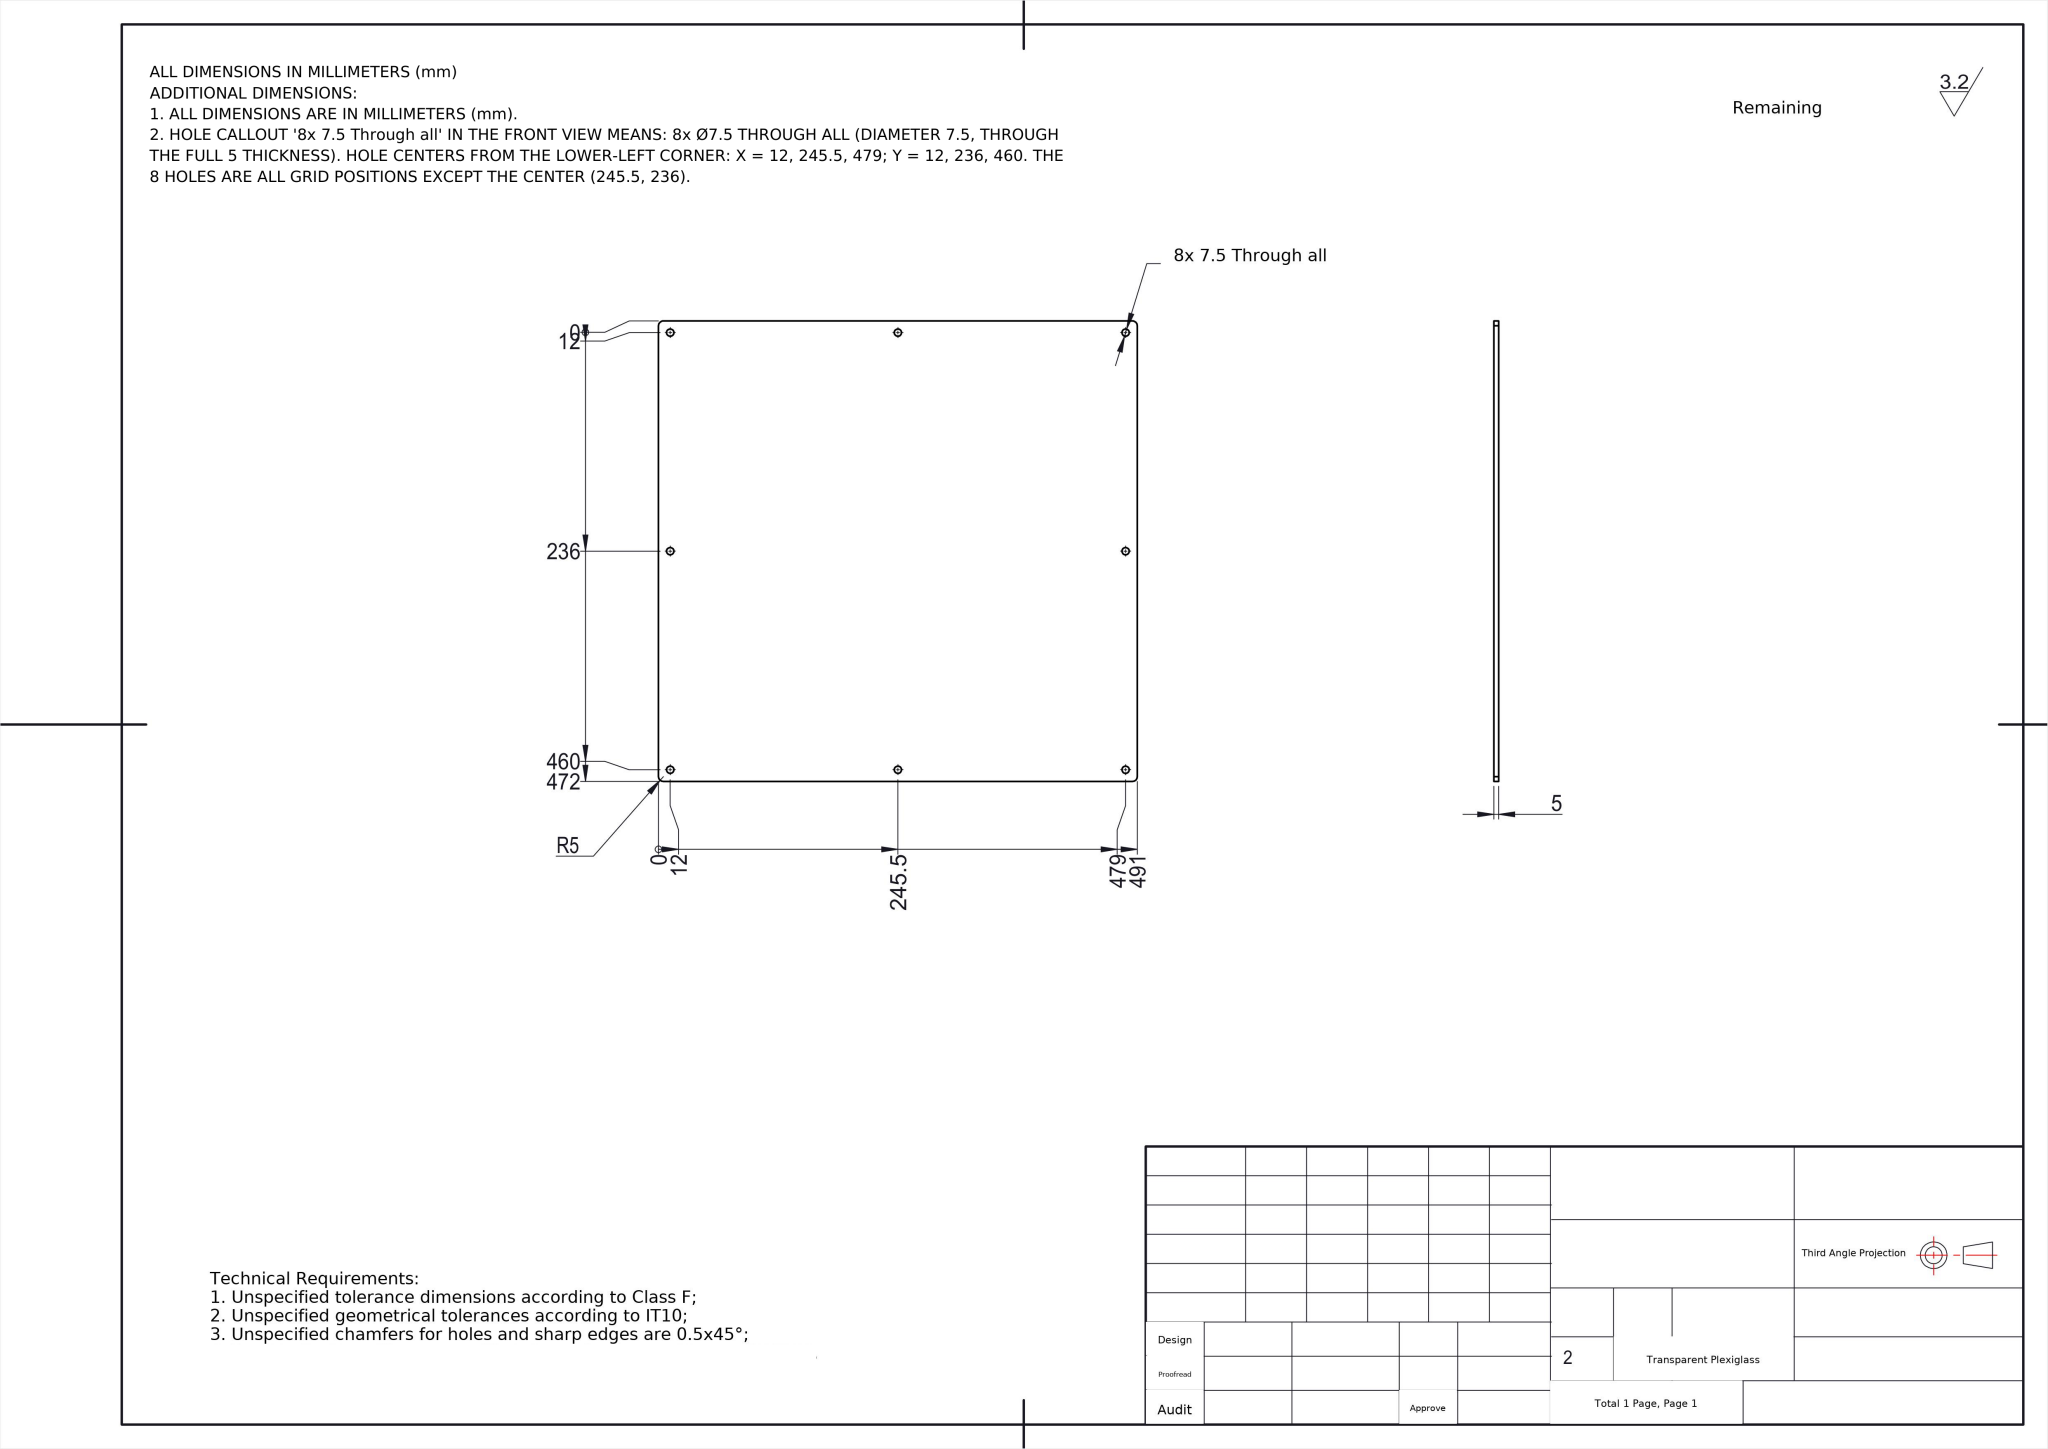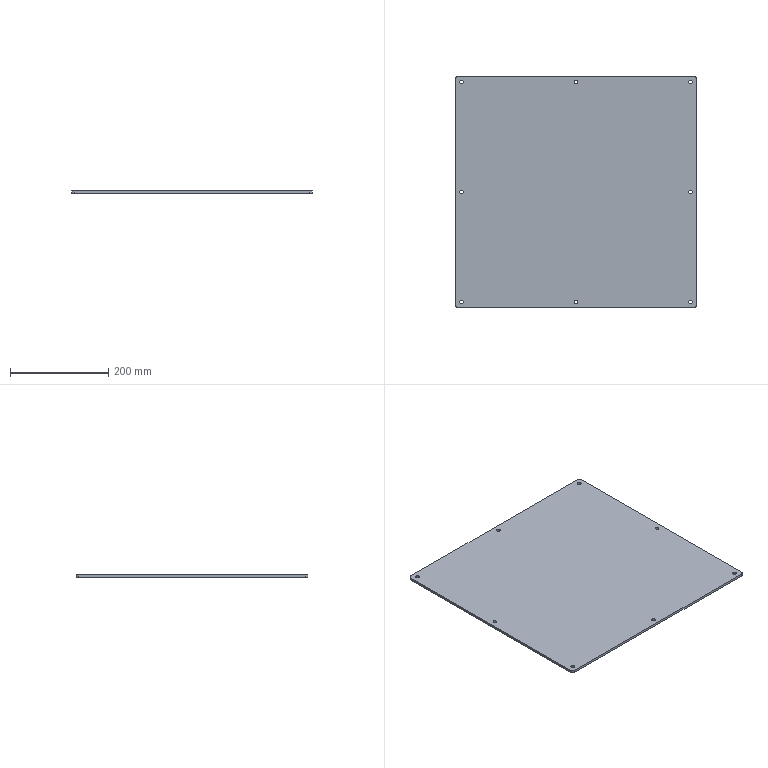Part | NX | mm | Square Eight-Hole Mounting Plate | 1 solid | 26 faces | box 491 x 472 x 5 mm | volume 1156886 mm3 | cylinder 20 | plane 6 | commonest cylinder face diameters 7.5 x16 10 x4